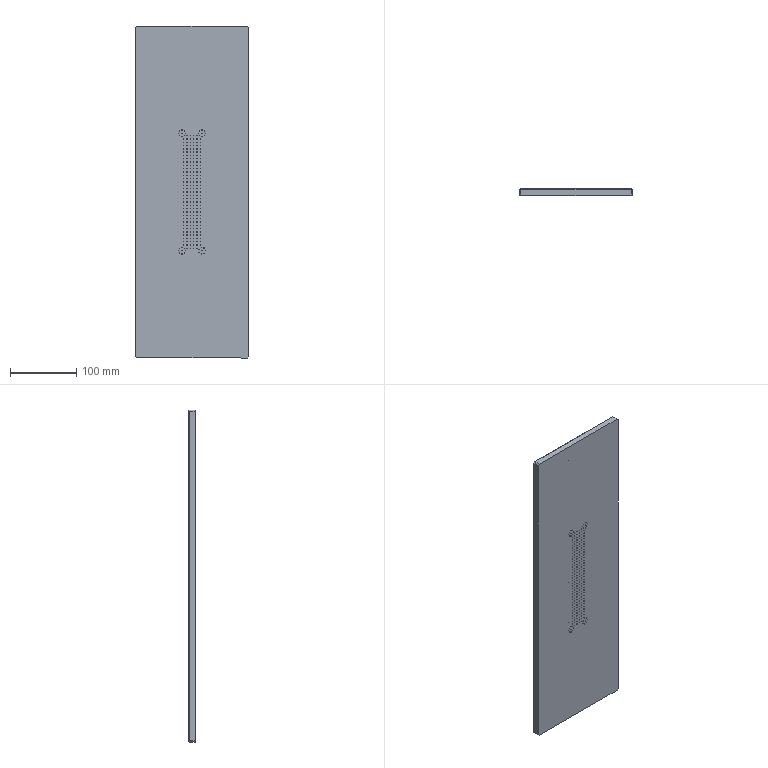Component | SolidWorks | 013-1 | 1 solid | 559 faces | volume 807313 mm3 | cylinder 512 | cone 24 | plane 23 | commonest cylinder face diameters 0.6 x482 3.3 x24 15 x6 | material AL6061